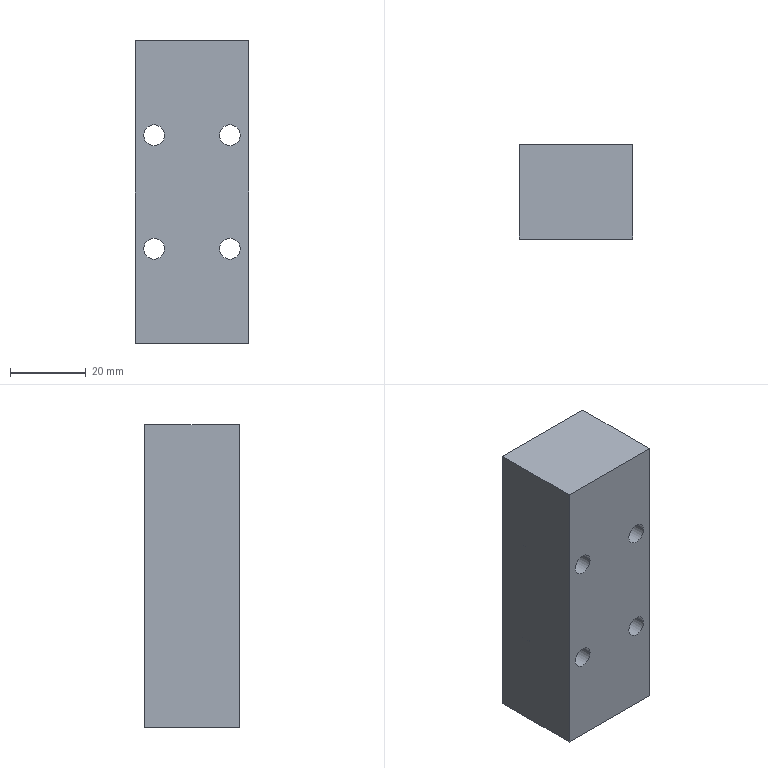Component | SolidWorks | CS021-A10-A027-1 | 1 solid | 42 faces | box 30 x 25 x 80 mm | volume 54829 mm3 | cylinder 24 | plane 10 | cone 8 | commonest cylinder face diameters 4.2 x8 9.5 x8 5.5 x8 | material AL6061
build123d program:
from build123d import *

# Parameters (mm, degrees)
SKETCH1_W                                          = 30
SKETCH1_H                                          = 80
BOSS_EXTRUDE1_DEPTH                                = 12.5
HOLE_SIZE_ACCORDING_TO_SLOTTED_PAN_HEA_D           = 5.5
HOLE_SIZE_ACCORDING_TO_SLOTTED_PAN_HEA_CBORE_D     = 9.5
HOLE_SIZE_ACCORDING_TO_SLOTTED_PAN_HEA_CBORE_DEPTH = 10
M5_TAPPED_HOLE2_D                                  = 4.2
M5_TAPPED_HOLE2_DEPTH                              = 16
M5_TAPPED_HOLE2_TIP                                = 1.262


with BuildPart() as part:
    # Sketch1 → Boss-Extrude1 (new, symmetric)
    with BuildSketch(Plane.XY):
        Rectangle(SKETCH1_W, SKETCH1_H)
    extrude(amount=BOSS_EXTRUDE1_DEPTH, both=True)

    # Hole Size _according to_ Slotted Pan Hea (through all)
    with Locations(Plane(origin=(0, 0, -12.5), x_dir=(-1, 0, 0), z_dir=(0, 0, -1))):
        with Locations((-10, 15), (10, 15), (10, -15), (-10, -15)):
            CounterBoreHole(HOLE_SIZE_ACCORDING_TO_SLOTTED_PAN_HEA_D / 2, HOLE_SIZE_ACCORDING_TO_SLOTTED_PAN_HEA_CBORE_D / 2, HOLE_SIZE_ACCORDING_TO_SLOTTED_PAN_HEA_CBORE_DEPTH)

    # M5 Tapped Hole2
    with Locations(Plane(origin=(0, 0, -12.5), x_dir=(-1, 0, 0), z_dir=(0, 0, -1))):
        with Locations((-9, 25), (9, 25), (9, -25), (-9, -25)):
            Hole(M5_TAPPED_HOLE2_D / 2, depth=M5_TAPPED_HOLE2_DEPTH)
            with Locations((0, 0, -(M5_TAPPED_HOLE2_DEPTH + M5_TAPPED_HOLE2_TIP / 2))):  # 118° drill point
                Cone(0, M5_TAPPED_HOLE2_D / 2, M5_TAPPED_HOLE2_TIP, mode=Mode.SUBTRACT)


solid = part.part

# Placed as in the assembly
solid = solid.moved(Location((152.449, 109.817, 0), (90, 0, 0)))